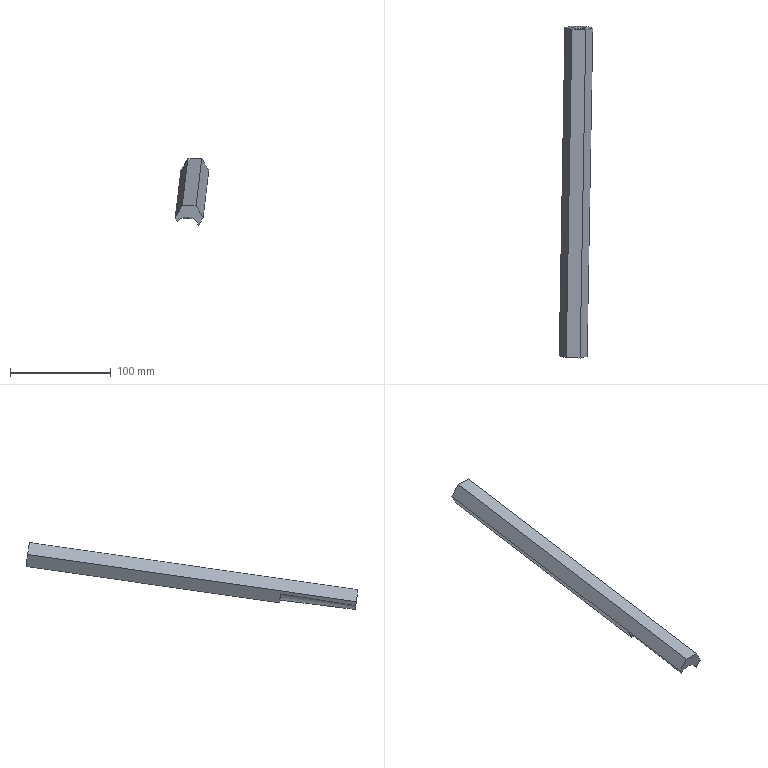Component | NX | HEX_STEEL | 1 solid | 12 faces | box 33.33 x 330.25 x 66.52 mm | volume 143704 mm3 | plane 9 | cylinder 2 | cone 1 | commonest cylinder face diameters 14 x1 25 x1
STEP:
#1=CARTESIAN_POINT('',(0.,0.,0.));
#2=DIRECTION('',(0.,0.,1.));
#3=DIRECTION('',(1.,0.,0.));
#4=AXIS2_PLACEMENT_3D('',#1,#2,#3);
#5=CARTESIAN_POINT('',(1340.241,698.717,571.115));
#6=VERTEX_POINT('',#5);
#7=CARTESIAN_POINT('',(1333.313,700.539,559.253));
#8=VERTEX_POINT('',#7);
#9=CARTESIAN_POINT('',(1340.241,698.717,571.115));
#10=DIRECTION('',(-0.4999,0.1315,-0.856));
#11=VECTOR('',#10,1.);
#12=LINE('',#9,#11);
#13=CARTESIAN_POINT('',(1345.864,1025.32,618.005));
#14=DIRECTION('',(-0.8659,-0.05645,0.497));
#15=DIRECTION('',(0.4978,0.,0.8673));
#16=AXIS2_PLACEMENT_3D('',#13,#14,#15);
#17=PLANE('',#16);
#18=CARTESIAN_POINT('',(-43.467,-327.125));
#19=DIRECTION('',(-0.9913,0.1317));
#20=VECTOR('',#19,1.);
#21=LINE('',#18,#20);
#22=(GEOMETRIC_REPRESENTATION_CONTEXT(2)PARAMETRIC_REPRESENTATION_CONTEXT()REPRESENTATION_CONTEXT('',''));
#23=DEFINITIONAL_REPRESENTATION('',(#21),#22);
#24=PCURVE('',#17,#23);
#25=CARTESIAN_POINT('',(13.556,791.589,83.34));
#26=DIRECTION('',(-0.01704,-0.9897,-0.1421));
#27=DIRECTION('',(0.,0.1421,-0.9899));
#28=AXIS2_PLACEMENT_3D('',#25,#26,#27);
#29=PLANE('',#28);
#30=CARTESIAN_POINT('',(-496.022,1326.877));
#31=DIRECTION('',(0.866,-0.5));
#32=VECTOR('',#31,1.);
#33=LINE('',#30,#32);
#34=(GEOMETRIC_REPRESENTATION_CONTEXT(2)PARAMETRIC_REPRESENTATION_CONTEXT()REPRESENTATION_CONTEXT('',''));
#35=DEFINITIONAL_REPRESENTATION('',(#33),#34);
#36=PCURVE('',#29,#35);
#37=SURFACE_CURVE('',#12,(#24,#36),.PCURVE_S1.);
#38=EDGE_CURVE('',#6,#8,#37,.T.);
#39=ORIENTED_EDGE('',*,*,#38,.F.);
#40=CARTESIAN_POINT('',(1345.864,1025.32,618.005));
#41=VERTEX_POINT('',#40);
#42=CARTESIAN_POINT('',(1345.864,1025.32,618.005));
#43=DIRECTION('',(-0.01704,-0.9897,-0.1421));
#44=VECTOR('',#43,1.);
#45=LINE('',#42,#44);
#46=CARTESIAN_POINT('',(0.,0.));
#47=DIRECTION('',(-0.1317,-0.9913));
#48=VECTOR('',#47,1.);
#49=LINE('',#46,#48);
#50=(GEOMETRIC_REPRESENTATION_CONTEXT(2)PARAMETRIC_REPRESENTATION_CONTEXT()REPRESENTATION_CONTEXT('',''));
#51=DEFINITIONAL_REPRESENTATION('',(#49),#50);
#52=PCURVE('',#17,#51);
#53=CARTESIAN_POINT('',(1359.718,1025.087,617.972));
#54=DIRECTION('',(0.,-0.1421,0.9899));
#55=DIRECTION('',(-0.,-0.9899,-0.1421));
#56=AXIS2_PLACEMENT_3D('',#53,#54,#55);
#57=PLANE('',#56);
#58=CARTESIAN_POINT('',(-0.2361,-13.854));
#59=DIRECTION('',(0.9999,-0.01704));
#60=VECTOR('',#59,1.);
#61=LINE('',#58,#60);
#62=(GEOMETRIC_REPRESENTATION_CONTEXT(2)PARAMETRIC_REPRESENTATION_CONTEXT()REPRESENTATION_CONTEXT('',''));
#63=DEFINITIONAL_REPRESENTATION('',(#61),#62);
#64=PCURVE('',#57,#63);
#65=SURFACE_CURVE('',#45,(#52,#64),.PCURVE_S1.);
#66=EDGE_CURVE('',#41,#6,#65,.T.);
#67=ORIENTED_EDGE('',*,*,#66,.F.);
#68=CARTESIAN_POINT('',(1338.937,1027.142,606.144));
#69=VERTEX_POINT('',#68);
#70=CARTESIAN_POINT('',(1345.864,1025.32,618.005));
#71=DIRECTION('',(-0.4999,0.1315,-0.856));
#72=VECTOR('',#71,1.);
#73=LINE('',#70,#72);
#74=CARTESIAN_POINT('',(0.,0.));
#75=DIRECTION('',(-0.9913,0.1317));
#76=VECTOR('',#75,1.);
#77=LINE('',#74,#76);
#78=(GEOMETRIC_REPRESENTATION_CONTEXT(2)PARAMETRIC_REPRESENTATION_CONTEXT()REPRESENTATION_CONTEXT('',''));
#79=DEFINITIONAL_REPRESENTATION('',(#77),#78);
#80=PCURVE('',#17,#79);
#81=CARTESIAN_POINT('',(19.179,1118.192,130.231));
#82=DIRECTION('',(-0.01704,-0.9897,-0.1421));
#83=DIRECTION('',(0.,0.1421,-0.9899));
#84=AXIS2_PLACEMENT_3D('',#81,#82,#83);
#85=PLANE('',#84);
#86=CARTESIAN_POINT('',(-496.022,1326.877));
#87=DIRECTION('',(0.866,-0.5));
#88=VECTOR('',#87,1.);
#89=LINE('',#86,#88);
#90=(GEOMETRIC_REPRESENTATION_CONTEXT(2)PARAMETRIC_REPRESENTATION_CONTEXT()REPRESENTATION_CONTEXT('',''));
#91=DEFINITIONAL_REPRESENTATION('',(#89),#90);
#92=PCURVE('',#85,#91);
#93=SURFACE_CURVE('',#73,(#80,#92),.PCURVE_S1.);
#94=EDGE_CURVE('',#41,#69,#93,.T.);
#95=ORIENTED_EDGE('',*,*,#94,.T.);
#96=CARTESIAN_POINT('',(1338.937,1027.142,606.144));
#97=DIRECTION('',(-0.01704,-0.9897,-0.1421));
#98=VECTOR('',#97,1.);
#99=LINE('',#96,#98);
#100=CARTESIAN_POINT('',(-13.736,1.825));
#101=DIRECTION('',(-0.1317,-0.9913));
#102=VECTOR('',#101,1.);
#103=LINE('',#100,#102);
#104=(GEOMETRIC_REPRESENTATION_CONTEXT(2)PARAMETRIC_REPRESENTATION_CONTEXT()REPRESENTATION_CONTEXT('',''));
#105=DEFINITIONAL_REPRESENTATION('',(#103),#104);
#106=PCURVE('',#17,#105);
#107=CARTESIAN_POINT('',(1338.937,1027.142,606.144));
#108=DIRECTION('',(-0.8659,0.08566,-0.4928));
#109=DIRECTION('',(-0.4946,0.,0.8691));
#110=AXIS2_PLACEMENT_3D('',#107,#108,#109);
#111=PLANE('',#110);
#112=CARTESIAN_POINT('',(0.,0.));
#113=DIRECTION('',(-0.1151,-0.9934));
#114=VECTOR('',#113,1.);
#115=LINE('',#112,#114);
#116=(GEOMETRIC_REPRESENTATION_CONTEXT(2)PARAMETRIC_REPRESENTATION_CONTEXT()REPRESENTATION_CONTEXT('',''));
#117=DEFINITIONAL_REPRESENTATION('',(#115),#116);
#118=PCURVE('',#111,#117);
#119=SURFACE_CURVE('',#99,(#106,#118),.PCURVE_S1.);
#120=EDGE_CURVE('',#69,#8,#119,.T.);
#121=ORIENTED_EDGE('',*,*,#120,.T.);
#122=EDGE_LOOP('',(#39,#67,#95,#121));
#123=FACE_BOUND('',#122,.T.);
#124=ADVANCED_FACE('',(#123),#17,.T.);
#125=CARTESIAN_POINT('',(1336.24,775.365,567.118));
#126=VERTEX_POINT('',#125);
#127=CARTESIAN_POINT('',(1341.524,776.666,558.06));
#128=VERTEX_POINT('',#127);
#129=CARTESIAN_POINT('',(1335.68,775.228,568.077));
#130=DIRECTION('',(0.5001,0.1231,-0.8572));
#131=VECTOR('',#130,1.);
#132=LINE('',#129,#131);
#133=CARTESIAN_POINT('',(-31.473,-252.844));
#134=DIRECTION('',(-0.9923,0.1235));
#135=VECTOR('',#134,1.);
#136=LINE('',#133,#135);
#137=(GEOMETRIC_REPRESENTATION_CONTEXT(2)PARAMETRIC_REPRESENTATION_CONTEXT()REPRESENTATION_CONTEXT('',''));
#138=DEFINITIONAL_REPRESENTATION('',(#136),#137);
#139=PCURVE('',#111,#138);
#140=CARTESIAN_POINT('',(1344.754,776.666,558.06));
#141=DIRECTION('',(0.,0.9899,0.1421));
#142=DIRECTION('',(0.,-0.1421,0.9899));
#143=AXIS2_PLACEMENT_3D('',#140,#141,#142);
#144=PLANE('',#143);
#145=CARTESIAN_POINT('',(10.12,-9.074));
#146=DIRECTION('',(-0.866,0.5001));
#147=VECTOR('',#146,1.);
#148=LINE('',#145,#147);
#149=(GEOMETRIC_REPRESENTATION_CONTEXT(2)PARAMETRIC_REPRESENTATION_CONTEXT()REPRESENTATION_CONTEXT('',''));
#150=DEFINITIONAL_REPRESENTATION('',(#148),#149);
#151=PCURVE('',#144,#150);
#152=SURFACE_CURVE('',#132,(#139,#151),.PCURVE_S1.);
#153=EDGE_CURVE('',#126,#128,#152,.T.);
#154=ORIENTED_EDGE('',*,*,#153,.F.);
#155=CARTESIAN_POINT('',(1335.433,701.025,555.614));
#156=VERTEX_POINT('',#155);
#157=CARTESIAN_POINT('',(1344.754,964.276,584.995));
#158=DIRECTION('',(-0.8659,0.08566,-0.4928));
#159=DIRECTION('',(0.01278,0.9887,0.1494));
#160=AXIS2_PLACEMENT_3D('',#157,#158,#159);
#161=ELLIPSE('',#160,847.024,12.5);
#162=CARTESIAN_POINT('',(-21.258,-63.098));
#163=DIRECTION('',(0.1235,0.9923));
#164=AXIS2_PLACEMENT_2D('',#162,#163);
#165=ELLIPSE('',#164,847.024,12.5);
#166=(GEOMETRIC_REPRESENTATION_CONTEXT(2)PARAMETRIC_REPRESENTATION_CONTEXT()REPRESENTATION_CONTEXT('',''));
#167=DEFINITIONAL_REPRESENTATION('',(#165),#166);
#168=PCURVE('',#111,#167);
#169=CARTESIAN_POINT('',(1344.754,657.884,541.006));
#170=DIRECTION('',(0.,0.9899,0.1421));
#171=DIRECTION('',(1.,0.,0.));
#172=AXIS2_PLACEMENT_3D('',#169,#170,#171);
#173=CYLINDRICAL_SURFACE('',#172,12.5);
#174=CARTESIAN_POINT('',(3.871,44.78));
#175=CARTESIAN_POINT('',(3.872,45.904));
#176=CARTESIAN_POINT('',(3.875,48.154));
#177=CARTESIAN_POINT('',(3.879,51.534));
#178=CARTESIAN_POINT('',(3.883,54.918));
#179=CARTESIAN_POINT('',(3.888,58.306));
#180=CARTESIAN_POINT('',(3.892,61.699));
#181=CARTESIAN_POINT('',(3.896,65.097));
#182=CARTESIAN_POINT('',(3.9,68.499));
#183=CARTESIAN_POINT('',(3.904,71.905));
#184=CARTESIAN_POINT('',(3.909,75.315));
#185=CARTESIAN_POINT('',(3.913,78.729));
#186=CARTESIAN_POINT('',(3.917,82.147));
#187=CARTESIAN_POINT('',(3.921,85.57));
#188=CARTESIAN_POINT('',(3.925,88.996));
#189=CARTESIAN_POINT('',(3.929,92.426));
#190=CARTESIAN_POINT('',(3.934,95.86));
#191=CARTESIAN_POINT('',(3.938,99.298));
#192=CARTESIAN_POINT('',(3.942,102.739));
#193=CARTESIAN_POINT('',(3.946,106.184));
#194=CARTESIAN_POINT('',(3.95,109.633));
#195=CARTESIAN_POINT('',(3.955,113.085));
#196=CARTESIAN_POINT('',(3.959,116.54));
#197=CARTESIAN_POINT('',(3.962,118.846));
#198=CARTESIAN_POINT('',(3.963,120.));
#199=B_SPLINE_CURVE_WITH_KNOTS('',3,(#174,#175,#176,#177,#178,#179,#180,#181,#182,#183,#184,#185,#186,#187,#188,#189,#190,#191,#192,#193,#194,#195,#196,#197,#198),.UNSPECIFIED.,.F.,.F.,(4,1,1,1,1,1,1,1,1,1,1,1,1,1,1,1,1,1,1,1,1,1,4),(4.394,4.399,4.403,4.407,4.411,4.415,4.42,4.424,4.428,4.432,4.436,4.441,4.445,4.449,4.453,4.457,4.462,4.466,4.47,4.474,4.478,4.482,4.487),.QUASI_UNIFORM_KNOTS.);
#200=(GEOMETRIC_REPRESENTATION_CONTEXT(2)PARAMETRIC_REPRESENTATION_CONTEXT()REPRESENTATION_CONTEXT('',''));
#201=DEFINITIONAL_REPRESENTATION('',(#199),#200);
#202=PCURVE('',#173,#201);
#203=SURFACE_CURVE('',#161,(#168,#202),.PCURVE_S1.);
#204=EDGE_CURVE('',#156,#126,#203,.T.);
#205=ORIENTED_EDGE('',*,*,#204,.F.);
#206=CARTESIAN_POINT('',(1333.313,700.539,559.253));
#207=DIRECTION('',(0.4999,0.1146,-0.8584));
#208=VECTOR('',#207,1.);
#209=LINE('',#206,#208);
#210=CARTESIAN_POINT('',(-37.97,-327.808));
#211=DIRECTION('',(-0.9934,0.1151));
#212=VECTOR('',#211,1.);
#213=LINE('',#210,#212);
#214=(GEOMETRIC_REPRESENTATION_CONTEXT(2)PARAMETRIC_REPRESENTATION_CONTEXT()REPRESENTATION_CONTEXT('',''));
#215=DEFINITIONAL_REPRESENTATION('',(#213),#214);
#216=PCURVE('',#111,#215);
#217=CARTESIAN_POINT('',(-484.022,1319.949));
#218=DIRECTION('',(0.866,0.5));
#219=VECTOR('',#218,1.);
#220=LINE('',#217,#219);
#221=(GEOMETRIC_REPRESENTATION_CONTEXT(2)PARAMETRIC_REPRESENTATION_CONTEXT()REPRESENTATION_CONTEXT('',''));
#222=DEFINITIONAL_REPRESENTATION('',(#220),#221);
#223=PCURVE('',#29,#222);
#224=SURFACE_CURVE('',#209,(#216,#223),.PCURVE_S1.);
#225=EDGE_CURVE('',#8,#156,#224,.T.);
#226=ORIENTED_EDGE('',*,*,#225,.F.);
#227=ORIENTED_EDGE('',*,*,#120,.F.);
#228=CARTESIAN_POINT('',(1345.864,1028.731,594.249));
#229=VERTEX_POINT('',#228);
#230=CARTESIAN_POINT('',(1338.937,1027.142,606.144));
#231=DIRECTION('',(0.4999,0.1146,-0.8584));
#232=VECTOR('',#231,1.);
#233=LINE('',#230,#232);
#234=CARTESIAN_POINT('',(0.,0.));
#235=DIRECTION('',(-0.9934,0.1151));
#236=VECTOR('',#235,1.);
#237=LINE('',#234,#236);
#238=(GEOMETRIC_REPRESENTATION_CONTEXT(2)PARAMETRIC_REPRESENTATION_CONTEXT()REPRESENTATION_CONTEXT('',''));
#239=DEFINITIONAL_REPRESENTATION('',(#237),#238);
#240=PCURVE('',#111,#239);
#241=CARTESIAN_POINT('',(-484.022,1319.949));
#242=DIRECTION('',(0.866,0.5));
#243=VECTOR('',#242,1.);
#244=LINE('',#241,#243);
#245=(GEOMETRIC_REPRESENTATION_CONTEXT(2)PARAMETRIC_REPRESENTATION_CONTEXT()REPRESENTATION_CONTEXT('',''));
#246=DEFINITIONAL_REPRESENTATION('',(#244),#245);
#247=PCURVE('',#85,#246);
#248=SURFACE_CURVE('',#233,(#240,#247),.PCURVE_S1.);
#249=EDGE_CURVE('',#69,#229,#248,.T.);
#250=ORIENTED_EDGE('',*,*,#249,.T.);
#251=CARTESIAN_POINT('',(1345.864,1028.731,594.249));
#252=DIRECTION('',(-0.01704,-0.9897,-0.1421));
#253=VECTOR('',#252,1.);
#254=LINE('',#251,#253);
#255=CARTESIAN_POINT('',(-13.764,1.594));
#256=DIRECTION('',(-0.1151,-0.9934));
#257=VECTOR('',#256,1.);
#258=LINE('',#255,#257);
#259=(GEOMETRIC_REPRESENTATION_CONTEXT(2)PARAMETRIC_REPRESENTATION_CONTEXT()REPRESENTATION_CONTEXT('',''));
#260=DEFINITIONAL_REPRESENTATION('',(#258),#259);
#261=PCURVE('',#111,#260);
#262=CARTESIAN_POINT('',(1345.864,1028.731,594.249));
#263=DIRECTION('',(-0.,0.1421,-0.9899));
#264=DIRECTION('',(0.,0.9899,0.1421));
#265=AXIS2_PLACEMENT_3D('',#262,#263,#264);
#266=PLANE('',#265);
#267=CARTESIAN_POINT('',(0.,0.));
#268=DIRECTION('',(-0.9999,-0.01704));
#269=VECTOR('',#268,1.);
#270=LINE('',#267,#269);
#271=(GEOMETRIC_REPRESENTATION_CONTEXT(2)PARAMETRIC_REPRESENTATION_CONTEXT()REPRESENTATION_CONTEXT('',''));
#272=DEFINITIONAL_REPRESENTATION('',(#270),#271);
#273=PCURVE('',#266,#272);
#274=SURFACE_CURVE('',#254,(#261,#273),.PCURVE_S1.);
#275=EDGE_CURVE('',#229,#128,#274,.T.);
#276=ORIENTED_EDGE('',*,*,#275,.T.);
#277=EDGE_LOOP('',(#154,#205,#226,#227,#250,#276));
#278=FACE_BOUND('',#277,.T.);
#279=ADVANCED_FACE('',(#278),#111,.T.);
#280=CARTESIAN_POINT('',(1355.382,776.666,558.06));
#281=VERTEX_POINT('',#280);
#282=CARTESIAN_POINT('',(1345.864,776.666,558.06));
#283=DIRECTION('',(1.,0.,-0.));
#284=VECTOR('',#283,1.);
#285=LINE('',#282,#284);
#286=CARTESIAN_POINT('',(-254.65,-0.));
#287=DIRECTION('',(-0.,1.));
#288=VECTOR('',#287,1.);
#289=LINE('',#286,#288);
#290=(GEOMETRIC_REPRESENTATION_CONTEXT(2)PARAMETRIC_REPRESENTATION_CONTEXT()REPRESENTATION_CONTEXT('',''));
#291=DEFINITIONAL_REPRESENTATION('',(#289),#290);
#292=PCURVE('',#266,#291);
#293=CARTESIAN_POINT('',(0.,1.11));
#294=DIRECTION('',(-0.,1.));
#295=VECTOR('',#294,1.);
#296=LINE('',#293,#295);
#297=(GEOMETRIC_REPRESENTATION_CONTEXT(2)PARAMETRIC_REPRESENTATION_CONTEXT()REPRESENTATION_CONTEXT('',''));
#298=DEFINITIONAL_REPRESENTATION('',(#296),#297);
#299=PCURVE('',#144,#298);
#300=SURFACE_CURVE('',#285,(#292,#299),.PCURVE_S1.);
#301=EDGE_CURVE('',#128,#281,#300,.T.);
#302=ORIENTED_EDGE('',*,*,#301,.F.);
#303=ORIENTED_EDGE('',*,*,#275,.F.);
#304=CARTESIAN_POINT('',(1359.718,1028.497,594.215));
#305=VERTEX_POINT('',#304);
#306=CARTESIAN_POINT('',(1345.864,1028.731,594.249));
#307=DIRECTION('',(0.9999,-0.01687,-0.002422));
#308=VECTOR('',#307,1.);
#309=LINE('',#306,#308);
#310=CARTESIAN_POINT('',(0.,0.));
#311=DIRECTION('',(-0.01704,0.9999));
#312=VECTOR('',#311,1.);
#313=LINE('',#310,#312);
#314=(GEOMETRIC_REPRESENTATION_CONTEXT(2)PARAMETRIC_REPRESENTATION_CONTEXT()REPRESENTATION_CONTEXT('',''));
#315=DEFINITIONAL_REPRESENTATION('',(#313),#314);
#316=PCURVE('',#266,#315);
#317=CARTESIAN_POINT('',(-472.022,1326.877));
#318=DIRECTION('',(0.,1.));
#319=VECTOR('',#318,1.);
#320=LINE('',#317,#319);
#321=(GEOMETRIC_REPRESENTATION_CONTEXT(2)PARAMETRIC_REPRESENTATION_CONTEXT()REPRESENTATION_CONTEXT('',''));
#322=DEFINITIONAL_REPRESENTATION('',(#320),#321);
#323=PCURVE('',#85,#322);
#324=SURFACE_CURVE('',#309,(#316,#323),.PCURVE_S1.);
#325=EDGE_CURVE('',#229,#305,#324,.T.);
#326=ORIENTED_EDGE('',*,*,#325,.T.);
#327=CARTESIAN_POINT('',(1359.718,1028.497,594.215));
#328=DIRECTION('',(-0.01704,-0.9897,-0.1421));
#329=VECTOR('',#328,1.);
#330=LINE('',#327,#329);
#331=CARTESIAN_POINT('',(-0.2361,13.854));
#332=DIRECTION('',(-0.9999,-0.01704));
#333=VECTOR('',#332,1.);
#334=LINE('',#331,#333);
#335=(GEOMETRIC_REPRESENTATION_CONTEXT(2)PARAMETRIC_REPRESENTATION_CONTEXT()REPRESENTATION_CONTEXT('',''));
#336=DEFINITIONAL_REPRESENTATION('',(#334),#335);
#337=PCURVE('',#266,#336);
#338=CARTESIAN_POINT('',(1359.718,1028.497,594.215));
#339=DIRECTION('',(0.8659,0.05645,-0.497));
#340=DIRECTION('',(-0.4978,0.,-0.8673));
#341=AXIS2_PLACEMENT_3D('',#338,#339,#340);
#342=PLANE('',#341);
#343=CARTESIAN_POINT('',(0.,0.));
#344=DIRECTION('',(0.1317,-0.9913));
#345=VECTOR('',#344,1.);
#346=LINE('',#343,#345);
#347=(GEOMETRIC_REPRESENTATION_CONTEXT(2)PARAMETRIC_REPRESENTATION_CONTEXT()REPRESENTATION_CONTEXT('',''));
#348=DEFINITIONAL_REPRESENTATION('',(#346),#347);
#349=PCURVE('',#342,#348);
#350=SURFACE_CURVE('',#330,(#337,#349),.PCURVE_S1.);
#351=EDGE_CURVE('',#305,#281,#350,.T.);
#352=ORIENTED_EDGE('',*,*,#351,.T.);
#353=EDGE_LOOP('',(#302,#303,#326,#352));
#354=FACE_BOUND('',#353,.T.);
#355=ADVANCED_FACE('',(#354),#266,.T.);
#356=CARTESIAN_POINT('',(1356.954,776.279,560.754));
#357=VERTEX_POINT('',#356);
#358=CARTESIAN_POINT('',(1356.467,776.399,559.918));
#359=DIRECTION('',(0.5001,-0.1231,0.8572));
#360=VECTOR('',#359,1.);
#361=LINE('',#358,#360);
#362=CARTESIAN_POINT('',(31.364,-252.501));
#363=DIRECTION('',(-0.9924,-0.1233));
#364=VECTOR('',#363,1.);
#365=LINE('',#362,#364);
#366=(GEOMETRIC_REPRESENTATION_CONTEXT(2)PARAMETRIC_REPRESENTATION_CONTEXT()REPRESENTATION_CONTEXT('',''));
#367=DEFINITIONAL_REPRESENTATION('',(#365),#366);
#368=PCURVE('',#342,#367);
#369=CARTESIAN_POINT('',(1.878,11.712));
#370=DIRECTION('',(0.866,0.5001));
#371=VECTOR('',#370,1.);
#372=LINE('',#369,#371);
#373=(GEOMETRIC_REPRESENTATION_CONTEXT(2)PARAMETRIC_REPRESENTATION_CONTEXT()REPRESENTATION_CONTEXT('',''));
#374=DEFINITIONAL_REPRESENTATION('',(#372),#373);
#375=PCURVE('',#144,#374);
#376=SURFACE_CURVE('',#361,(#368,#375),.PCURVE_S1.);
#377=EDGE_CURVE('',#281,#357,#376,.T.);
#378=ORIENTED_EDGE('',*,*,#377,.F.);
#379=ORIENTED_EDGE('',*,*,#351,.F.);
#380=CARTESIAN_POINT('',(1366.646,1026.675,606.077));
#381=VERTEX_POINT('',#380);
#382=CARTESIAN_POINT('',(1359.718,1028.497,594.215));
#383=DIRECTION('',(0.4999,-0.1315,0.856));
#384=VECTOR('',#383,1.);
#385=LINE('',#382,#384);
#386=CARTESIAN_POINT('',(0.,0.));
#387=DIRECTION('',(-0.9913,-0.1317));
#388=VECTOR('',#387,1.);
#389=LINE('',#386,#388);
#390=(GEOMETRIC_REPRESENTATION_CONTEXT(2)PARAMETRIC_REPRESENTATION_CONTEXT()REPRESENTATION_CONTEXT('',''));
#391=DEFINITIONAL_REPRESENTATION('',(#389),#390);
#392=PCURVE('',#342,#391);
#393=CARTESIAN_POINT('',(-472.022,1340.734));
#394=DIRECTION('',(-0.866,0.5));
#395=VECTOR('',#394,1.);
#396=LINE('',#393,#395);
#397=(GEOMETRIC_REPRESENTATION_CONTEXT(2)PARAMETRIC_REPRESENTATION_CONTEXT()REPRESENTATION_CONTEXT('',''));
#398=DEFINITIONAL_REPRESENTATION('',(#396),#397);
#399=PCURVE('',#85,#398);
#400=SURFACE_CURVE('',#385,(#392,#399),.PCURVE_S1.);
#401=EDGE_CURVE('',#305,#381,#400,.T.);
#402=ORIENTED_EDGE('',*,*,#401,.T.);
#403=CARTESIAN_POINT('',(1361.022,700.072,559.186));
#404=VERTEX_POINT('',#403);
#405=CARTESIAN_POINT('',(1366.646,1026.675,606.077));
#406=DIRECTION('',(-0.01704,-0.9897,-0.1421));
#407=VECTOR('',#406,1.);
#408=LINE('',#405,#407);
#409=CARTESIAN_POINT('',(-13.736,-1.825));
#410=DIRECTION('',(0.1317,-0.9913));
#411=VECTOR('',#410,1.);
#412=LINE('',#409,#411);
#413=(GEOMETRIC_REPRESENTATION_CONTEXT(2)PARAMETRIC_REPRESENTATION_CONTEXT()REPRESENTATION_CONTEXT('',''));
#414=DEFINITIONAL_REPRESENTATION('',(#412),#413);
#415=PCURVE('',#342,#414);
#416=CARTESIAN_POINT('',(1366.646,1026.675,606.077));
#417=DIRECTION('',(0.8659,-0.08566,0.4928));
#418=DIRECTION('',(0.4946,0.,-0.8691));
#419=AXIS2_PLACEMENT_3D('',#416,#417,#418);
#420=PLANE('',#419);
#421=CARTESIAN_POINT('',(0.,0.));
#422=DIRECTION('',(0.1151,-0.9934));
#423=VECTOR('',#422,1.);
#424=LINE('',#421,#423);
#425=(GEOMETRIC_REPRESENTATION_CONTEXT(2)PARAMETRIC_REPRESENTATION_CONTEXT()REPRESENTATION_CONTEXT('',''));
#426=DEFINITIONAL_REPRESENTATION('',(#424),#425);
#427=PCURVE('',#420,#426);
#428=SURFACE_CURVE('',#408,(#415,#427),.PCURVE_S1.);
#429=EDGE_CURVE('',#381,#404,#428,.T.);
#430=ORIENTED_EDGE('',*,*,#429,.T.);
#431=CARTESIAN_POINT('',(1356.524,701.255,551.485));
#432=VERTEX_POINT('',#431);
#433=CARTESIAN_POINT('',(1354.095,701.894,547.325));
#434=DIRECTION('',(0.4999,-0.1315,0.856));
#435=VECTOR('',#434,1.);
#436=LINE('',#433,#435);
#437=CARTESIAN_POINT('',(43.467,-327.125));
#438=DIRECTION('',(-0.9913,-0.1317));
#439=VECTOR('',#438,1.);
#440=LINE('',#437,#439);
#441=(GEOMETRIC_REPRESENTATION_CONTEXT(2)PARAMETRIC_REPRESENTATION_CONTEXT()REPRESENTATION_CONTEXT('',''));
#442=DEFINITIONAL_REPRESENTATION('',(#440),#441);
#443=PCURVE('',#342,#442);
#444=CARTESIAN_POINT('',(-472.022,1340.734));
#445=DIRECTION('',(-0.866,0.5));
#446=VECTOR('',#445,1.);
#447=LINE('',#444,#446);
#448=(GEOMETRIC_REPRESENTATION_CONTEXT(2)PARAMETRIC_REPRESENTATION_CONTEXT()REPRESENTATION_CONTEXT('',''));
#449=DEFINITIONAL_REPRESENTATION('',(#447),#448);
#450=PCURVE('',#29,#449);
#451=SURFACE_CURVE('',#436,(#443,#450),.PCURVE_S1.);
#452=EDGE_CURVE('',#432,#404,#451,.T.);
#453=ORIENTED_EDGE('',*,*,#452,.F.);
#454=CARTESIAN_POINT('',(1344.754,159.386,469.437));
#455=DIRECTION('',(0.8659,0.05645,-0.497));
#456=DIRECTION('',(0.01278,0.9908,0.1348));
#457=AXIS2_PLACEMENT_3D('',#454,#455,#456);
#458=ELLIPSE('',#457,847.024,12.5);
#459=CARTESIAN_POINT('',(115.667,-870.499));
#460=DIRECTION('',(-0.1233,0.9924));
#461=AXIS2_PLACEMENT_2D('',#459,#460);
#462=ELLIPSE('',#461,847.024,12.5);
#463=(GEOMETRIC_REPRESENTATION_CONTEXT(2)PARAMETRIC_REPRESENTATION_CONTEXT()REPRESENTATION_CONTEXT('',''));
#464=DEFINITIONAL_REPRESENTATION('',(#462),#463);
#465=PCURVE('',#342,#464);
#466=CARTESIAN_POINT('',(6.064,120.));
#467=CARTESIAN_POINT('',(6.062,118.924));
#468=CARTESIAN_POINT('',(6.058,116.767));
#469=CARTESIAN_POINT('',(6.052,113.511));
#470=CARTESIAN_POINT('',(6.047,110.235));
#471=CARTESIAN_POINT('',(6.041,106.94));
#472=CARTESIAN_POINT('',(6.036,103.626));
#473=CARTESIAN_POINT('',(6.03,100.292));
#474=CARTESIAN_POINT('',(6.024,96.939));
#475=CARTESIAN_POINT('',(6.019,93.567));
#476=CARTESIAN_POINT('',(6.013,90.176));
#477=CARTESIAN_POINT('',(6.007,86.767));
#478=CARTESIAN_POINT('',(6.002,83.338));
#479=CARTESIAN_POINT('',(5.996,79.892));
#480=CARTESIAN_POINT('',(5.99,76.426));
#481=CARTESIAN_POINT('',(5.985,72.942));
#482=CARTESIAN_POINT('',(5.979,69.44));
#483=CARTESIAN_POINT('',(5.974,65.92));
#484=CARTESIAN_POINT('',(5.968,62.382));
#485=CARTESIAN_POINT('',(5.962,58.825));
#486=CARTESIAN_POINT('',(5.957,55.251));
#487=CARTESIAN_POINT('',(5.951,51.659));
#488=CARTESIAN_POINT('',(5.945,48.05));
#489=CARTESIAN_POINT('',(5.942,45.632));
#490=CARTESIAN_POINT('',(5.94,44.42));
#491=B_SPLINE_CURVE_WITH_KNOTS('',3,(#466,#467,#468,#469,#470,#471,#472,#473,#474,#475,#476,#477,#478,#479,#480,#481,#482,#483,#484,#485,#486,#487,#488,#489,#490),.UNSPECIFIED.,.F.,.F.,(4,1,1,1,1,1,1,1,1,1,1,1,1,1,1,1,1,1,1,1,1,1,4),(0.7432,0.7488,0.7544,0.7601,0.7657,0.7713,0.777,0.7826,0.7882,0.7939,0.7995,0.8051,0.8108,0.8164,0.822,0.8276,0.8333,0.8389,0.8445,0.8502,0.8558,0.8614,0.8671),.QUASI_UNIFORM_KNOTS.);
#492=(GEOMETRIC_REPRESENTATION_CONTEXT(2)PARAMETRIC_REPRESENTATION_CONTEXT()REPRESENTATION_CONTEXT('',''));
#493=DEFINITIONAL_REPRESENTATION('',(#491),#492);
#494=PCURVE('',#173,#493);
#495=SURFACE_CURVE('',#458,(#465,#494),.PCURVE_S1.);
#496=EDGE_CURVE('',#357,#432,#495,.T.);
#497=ORIENTED_EDGE('',*,*,#496,.F.);
#498=EDGE_LOOP('',(#378,#379,#402,#430,#453,#497));
#499=FACE_BOUND('',#498,.T.);
#500=ADVANCED_FACE('',(#499),#342,.T.);
#501=CARTESIAN_POINT('',(1354.095,698.483,571.081));
#502=VERTEX_POINT('',#501);
#503=CARTESIAN_POINT('',(1361.022,700.072,559.186));
#504=DIRECTION('',(-0.4999,-0.1146,0.8584));
#505=VECTOR('',#504,1.);
#506=LINE('',#503,#505);
#507=CARTESIAN_POINT('',(37.97,-327.808));
#508=DIRECTION('',(-0.9934,-0.1151));
#509=VECTOR('',#508,1.);
#510=LINE('',#507,#509);
#511=(GEOMETRIC_REPRESENTATION_CONTEXT(2)PARAMETRIC_REPRESENTATION_CONTEXT()REPRESENTATION_CONTEXT('',''));
#512=DEFINITIONAL_REPRESENTATION('',(#510),#511);
#513=PCURVE('',#420,#512);
#514=CARTESIAN_POINT('',(-484.022,1347.662));
#515=DIRECTION('',(-0.866,-0.5));
#516=VECTOR('',#515,1.);
#517=LINE('',#514,#516);
#518=(GEOMETRIC_REPRESENTATION_CONTEXT(2)PARAMETRIC_REPRESENTATION_CONTEXT()REPRESENTATION_CONTEXT('',''));
#519=DEFINITIONAL_REPRESENTATION('',(#517),#518);
#520=PCURVE('',#29,#519);
#521=SURFACE_CURVE('',#506,(#513,#520),.PCURVE_S1.);
#522=EDGE_CURVE('',#404,#502,#521,.T.);
#523=ORIENTED_EDGE('',*,*,#522,.F.);
#524=ORIENTED_EDGE('',*,*,#429,.F.);
#525=CARTESIAN_POINT('',(1359.718,1025.087,617.972));
#526=VERTEX_POINT('',#525);
#527=CARTESIAN_POINT('',(1366.646,1026.675,606.077));
#528=DIRECTION('',(-0.4999,-0.1146,0.8584));
#529=VECTOR('',#528,1.);
#530=LINE('',#527,#529);
#531=CARTESIAN_POINT('',(0.,0.));
#532=DIRECTION('',(-0.9934,-0.1151));
#533=VECTOR('',#532,1.);
#534=LINE('',#531,#533);
#535=(GEOMETRIC_REPRESENTATION_CONTEXT(2)PARAMETRIC_REPRESENTATION_CONTEXT()REPRESENTATION_CONTEXT('',''));
#536=DEFINITIONAL_REPRESENTATION('',(#534),#535);
#537=PCURVE('',#420,#536);
#538=CARTESIAN_POINT('',(-484.022,1347.662));
#539=DIRECTION('',(-0.866,-0.5));
#540=VECTOR('',#539,1.);
#541=LINE('',#538,#540);
#542=(GEOMETRIC_REPRESENTATION_CONTEXT(2)PARAMETRIC_REPRESENTATION_CONTEXT()REPRESENTATION_CONTEXT('',''));
#543=DEFINITIONAL_REPRESENTATION('',(#541),#542);
#544=PCURVE('',#85,#543);
#545=SURFACE_CURVE('',#530,(#537,#544),.PCURVE_S1.);
#546=EDGE_CURVE('',#381,#526,#545,.T.);
#547=ORIENTED_EDGE('',*,*,#546,.T.);
#548=CARTESIAN_POINT('',(1359.718,1025.087,617.972));
#549=DIRECTION('',(-0.01704,-0.9897,-0.1421));
#550=VECTOR('',#549,1.);
#551=LINE('',#548,#550);
#552=CARTESIAN_POINT('',(-13.764,-1.594));
#553=DIRECTION('',(0.1151,-0.9934));
#554=VECTOR('',#553,1.);
#555=LINE('',#552,#554);
#556=(GEOMETRIC_REPRESENTATION_CONTEXT(2)PARAMETRIC_REPRESENTATION_CONTEXT()REPRESENTATION_CONTEXT('',''));
#557=DEFINITIONAL_REPRESENTATION('',(#555),#556);
#558=PCURVE('',#420,#557);
#559=CARTESIAN_POINT('',(0.,0.));
#560=DIRECTION('',(0.9999,-0.01704));
#561=VECTOR('',#560,1.);
#562=LINE('',#559,#561);
#563=(GEOMETRIC_REPRESENTATION_CONTEXT(2)PARAMETRIC_REPRESENTATION_CONTEXT()REPRESENTATION_CONTEXT('',''));
#564=DEFINITIONAL_REPRESENTATION('',(#562),#563);
#565=PCURVE('',#57,#564);
#566=SURFACE_CURVE('',#551,(#558,#565),.PCURVE_S1.);
#567=EDGE_CURVE('',#526,#502,#566,.T.);
#568=ORIENTED_EDGE('',*,*,#567,.T.);
#569=EDGE_LOOP('',(#523,#524,#547,#568));
#570=FACE_BOUND('',#569,.T.);
#571=ADVANCED_FACE('',(#570),#420,.T.);
#572=CARTESIAN_POINT('',(1354.095,698.483,571.081));
#573=DIRECTION('',(-0.9999,0.01687,0.002422));
#574=VECTOR('',#573,1.);
#575=LINE('',#572,#574);
#576=CARTESIAN_POINT('',(329.952,-5.623));
#577=DIRECTION('',(-0.01704,-0.9999));
#578=VECTOR('',#577,1.);
#579=LINE('',#576,#578);
#580=(GEOMETRIC_REPRESENTATION_CONTEXT(2)PARAMETRIC_REPRESENTATION_CONTEXT()REPRESENTATION_CONTEXT('',''));
#581=DEFINITIONAL_REPRESENTATION('',(#579),#580);
#582=PCURVE('',#57,#581);
#583=CARTESIAN_POINT('',(-496.022,1340.734));
#584=DIRECTION('',(-0.,-1.));
#585=VECTOR('',#584,1.);
#586=LINE('',#583,#585);
#587=(GEOMETRIC_REPRESENTATION_CONTEXT(2)PARAMETRIC_REPRESENTATION_CONTEXT()REPRESENTATION_CONTEXT('',''));
#588=DEFINITIONAL_REPRESENTATION('',(#586),#587);
#589=PCURVE('',#29,#588);
#590=SURFACE_CURVE('',#575,(#582,#589),.PCURVE_S1.);
#591=EDGE_CURVE('',#502,#6,#590,.T.);
#592=ORIENTED_EDGE('',*,*,#591,.F.);
#593=ORIENTED_EDGE('',*,*,#567,.F.);
#594=CARTESIAN_POINT('',(1359.718,1025.087,617.972));
#595=DIRECTION('',(-0.9999,0.01687,0.002422));
#596=VECTOR('',#595,1.);
#597=LINE('',#594,#596);
#598=CARTESIAN_POINT('',(0.,0.));
#599=DIRECTION('',(-0.01704,-0.9999));
#600=VECTOR('',#599,1.);
#601=LINE('',#598,#600);
#602=(GEOMETRIC_REPRESENTATION_CONTEXT(2)PARAMETRIC_REPRESENTATION_CONTEXT()REPRESENTATION_CONTEXT('',''));
#603=DEFINITIONAL_REPRESENTATION('',(#601),#602);
#604=PCURVE('',#57,#603);
#605=CARTESIAN_POINT('',(-496.022,1340.734));
#606=DIRECTION('',(-0.,-1.));
#607=VECTOR('',#606,1.);
#608=LINE('',#605,#607);
#609=(GEOMETRIC_REPRESENTATION_CONTEXT(2)PARAMETRIC_REPRESENTATION_CONTEXT()REPRESENTATION_CONTEXT('',''));
#610=DEFINITIONAL_REPRESENTATION('',(#608),#609);
#611=PCURVE('',#85,#610);
#612=SURFACE_CURVE('',#597,(#604,#611),.PCURVE_S1.);
#613=EDGE_CURVE('',#526,#41,#612,.T.);
#614=ORIENTED_EDGE('',*,*,#613,.T.);
#615=ORIENTED_EDGE('',*,*,#66,.T.);
#616=EDGE_LOOP('',(#592,#593,#614,#615));
#617=FACE_BOUND('',#616,.T.);
#618=ADVANCED_FACE('',(#617),#57,.T.);
#619=CARTESIAN_POINT('',(1352.791,1027.904,599.181));
#620=VERTEX_POINT('',#619);
#621=CARTESIAN_POINT('',(1352.791,1026.909,606.11));
#622=DIRECTION('',(-0.01704,-0.9897,-0.1421));
#623=DIRECTION('',(-0.,0.1421,-0.9899));
#624=AXIS2_PLACEMENT_3D('',#621,#622,#623);
#625=CIRCLE('',#624,7.);
#626=CARTESIAN_POINT('',(-484.022,1333.805));
#627=DIRECTION('',(1.,-0.));
#628=AXIS2_PLACEMENT_2D('',#626,#627);
#629=CIRCLE('',#628,7.);
#630=(GEOMETRIC_REPRESENTATION_CONTEXT(2)PARAMETRIC_REPRESENTATION_CONTEXT()REPRESENTATION_CONTEXT('',''));
#631=DEFINITIONAL_REPRESENTATION('',(#629),#630);
#632=PCURVE('',#85,#631);
#633=CARTESIAN_POINT('',(1352.791,1026.909,606.11));
#634=DIRECTION('',(-0.01704,-0.9897,-0.1421));
#635=DIRECTION('',(-0.,0.1421,-0.9899));
#636=AXIS2_PLACEMENT_3D('',#633,#634,#635);
#637=CYLINDRICAL_SURFACE('',#636,7.);
#638=CARTESIAN_POINT('',(0.,0.));
#639=DIRECTION('',(1.,0.));
#640=VECTOR('',#639,1.);
#641=LINE('',#638,#640);
#642=(GEOMETRIC_REPRESENTATION_CONTEXT(2)PARAMETRIC_REPRESENTATION_CONTEXT()REPRESENTATION_CONTEXT('',''));
#643=DEFINITIONAL_REPRESENTATION('',(#641),#642);
#644=PCURVE('',#637,#643);
#645=SURFACE_CURVE('',#625,(#632,#644),.PCURVE_S1.);
#646=EDGE_CURVE('',#620,#620,#645,.T.);
#647=ORIENTED_EDGE('',*,*,#646,.T.);
#648=EDGE_LOOP('',(#647));
#649=FACE_BOUND('',#648,.T.);
#650=ORIENTED_EDGE('',*,*,#94,.F.);
#651=ORIENTED_EDGE('',*,*,#613,.F.);
#652=ORIENTED_EDGE('',*,*,#546,.F.);
#653=ORIENTED_EDGE('',*,*,#401,.F.);
#654=ORIENTED_EDGE('',*,*,#325,.F.);
#655=ORIENTED_EDGE('',*,*,#249,.F.);
#656=EDGE_LOOP('',(#650,#651,#652,#653,#654,#655));
#657=FACE_BOUND('',#656,.T.);
#658=ADVANCED_FACE('',(#649,#657),#85,.F.);
#659=CARTESIAN_POINT('',(1344.754,702.052,547.347));
#660=DIRECTION('',(-0.01704,-0.9897,-0.1421));
#661=DIRECTION('',(-0.9999,0.01687,0.002422));
#662=AXIS2_PLACEMENT_3D('',#659,#660,#661);
#663=ELLIPSE('',#662,12.502,12.5);
#664=CARTESIAN_POINT('',(-472.022,1331.391));
#665=DIRECTION('',(0.,-1.));
#666=AXIS2_PLACEMENT_2D('',#664,#665);
#667=ELLIPSE('',#666,12.502,12.5);
#668=(GEOMETRIC_REPRESENTATION_CONTEXT(2)PARAMETRIC_REPRESENTATION_CONTEXT()REPRESENTATION_CONTEXT('',''));
#669=DEFINITIONAL_REPRESENTATION('',(#667),#668);
#670=PCURVE('',#29,#669);
#671=CARTESIAN_POINT('',(5.94,44.42));
#672=CARTESIAN_POINT('',(3.871,44.78));
#673=B_SPLINE_CURVE_WITH_KNOTS('',1,(#671,#672),.UNSPECIFIED.,.F.,.F.,(2,2),(3.485,5.554),.PIECEWISE_BEZIER_KNOTS.);
#674=(GEOMETRIC_REPRESENTATION_CONTEXT(2)PARAMETRIC_REPRESENTATION_CONTEXT()REPRESENTATION_CONTEXT('',''));
#675=DEFINITIONAL_REPRESENTATION('',(#673),#674);
#676=PCURVE('',#173,#675);
#677=SURFACE_CURVE('',#663,(#670,#676),.PCURVE_S1.);
#678=EDGE_CURVE('',#432,#156,#677,.T.);
#679=ORIENTED_EDGE('',*,*,#678,.F.);
#680=ORIENTED_EDGE('',*,*,#452,.T.);
#681=ORIENTED_EDGE('',*,*,#522,.T.);
#682=ORIENTED_EDGE('',*,*,#591,.T.);
#683=ORIENTED_EDGE('',*,*,#38,.T.);
#684=ORIENTED_EDGE('',*,*,#225,.T.);
#685=EDGE_LOOP('',(#679,#680,#681,#682,#683,#684));
#686=FACE_BOUND('',#685,.T.);
#687=ADVANCED_FACE('',(#686),#29,.T.);
#688=CARTESIAN_POINT('',(1352.144,988.305,607.64));
#689=VERTEX_POINT('',#688);
#690=CARTESIAN_POINT('',(1352.144,990.295,593.782));
#691=VERTEX_POINT('',#690);
#692=CARTESIAN_POINT('',(1352.144,989.3,600.711));
#693=DIRECTION('',(0.01704,0.9897,0.1421));
#694=DIRECTION('',(-0.,0.1421,-0.9899));
#695=AXIS2_PLACEMENT_3D('',#692,#693,#694);
#696=CIRCLE('',#695,7.);
#697=CARTESIAN_POINT('',(1352.144,989.3,600.711));
#698=DIRECTION('',(0.01704,0.9897,0.1421));
#699=DIRECTION('',(-0.,-0.1421,0.9899));
#700=AXIS2_PLACEMENT_3D('',#697,#698,#699);
#701=CONICAL_SURFACE('',#700,7.,1.047);
#702=CARTESIAN_POINT('',(-3.142,0.));
#703=DIRECTION('',(1.,0.));
#704=VECTOR('',#703,1.);
#705=LINE('',#702,#704);
#706=(GEOMETRIC_REPRESENTATION_CONTEXT(2)PARAMETRIC_REPRESENTATION_CONTEXT()REPRESENTATION_CONTEXT('',''));
#707=DEFINITIONAL_REPRESENTATION('',(#705),#706);
#708=PCURVE('',#701,#707);
#709=CARTESIAN_POINT('',(6.283,38.));
#710=DIRECTION('',(-1.,0.));
#711=VECTOR('',#710,1.);
#712=LINE('',#709,#711);
#713=(GEOMETRIC_REPRESENTATION_CONTEXT(2)PARAMETRIC_REPRESENTATION_CONTEXT()REPRESENTATION_CONTEXT('',''));
#714=DEFINITIONAL_REPRESENTATION('',(#712),#713);
#715=PCURVE('',#637,#714);
#716=SURFACE_CURVE('',#696,(#708,#715),.PCURVE_S1.);
#717=EDGE_CURVE('',#689,#691,#716,.T.);
#718=ORIENTED_EDGE('',*,*,#717,.F.);
#719=CARTESIAN_POINT('',(1352.075,985.3,600.136));
#720=VERTEX_POINT('',#719);
#721=CARTESIAN_POINT('',(1352.075,985.3,600.136));
#722=CARTESIAN_POINT('',(1352.144,988.305,607.64));
#723=B_SPLINE_CURVE_WITH_KNOTS('',1,(#721,#722),.UNSPECIFIED.,.F.,.F.,(2,2),(-8.083,0.),.PIECEWISE_BEZIER_KNOTS.);
#724=CARTESIAN_POINT('',(0.,0.));
#725=DIRECTION('',(0.,1.));
#726=VECTOR('',#725,1.);
#727=LINE('',#724,#726);
#728=(GEOMETRIC_REPRESENTATION_CONTEXT(2)PARAMETRIC_REPRESENTATION_CONTEXT()REPRESENTATION_CONTEXT('',''));
#729=DEFINITIONAL_REPRESENTATION('',(#727),#728);
#730=PCURVE('',#701,#729);
#731=CARTESIAN_POINT('',(6.283,0.));
#732=DIRECTION('',(0.,1.));
#733=VECTOR('',#732,1.);
#734=LINE('',#731,#733);
#735=(GEOMETRIC_REPRESENTATION_CONTEXT(2)PARAMETRIC_REPRESENTATION_CONTEXT()REPRESENTATION_CONTEXT('',''));
#736=DEFINITIONAL_REPRESENTATION('',(#734),#735);
#737=PCURVE('',#701,#736);
#738=SEAM_CURVE('',#723,(#730,#737),.PCURVE_S1.);
#739=EDGE_CURVE('',#720,#689,#738,.T.);
#740=ORIENTED_EDGE('',*,*,#739,.F.);
#741=ORIENTED_EDGE('',*,*,#739,.T.);
#742=CARTESIAN_POINT('',(1352.144,989.3,600.711));
#743=DIRECTION('',(0.01704,0.9897,0.1421));
#744=DIRECTION('',(-0.,0.1421,-0.9899));
#745=AXIS2_PLACEMENT_3D('',#742,#743,#744);
#746=CIRCLE('',#745,7.);
#747=CARTESIAN_POINT('',(3.142,0.));
#748=DIRECTION('',(1.,0.));
#749=VECTOR('',#748,1.);
#750=LINE('',#747,#749);
#751=(GEOMETRIC_REPRESENTATION_CONTEXT(2)PARAMETRIC_REPRESENTATION_CONTEXT()REPRESENTATION_CONTEXT('',''));
#752=DEFINITIONAL_REPRESENTATION('',(#750),#751);
#753=PCURVE('',#701,#752);
#754=CARTESIAN_POINT('',(6.283,38.));
#755=DIRECTION('',(-1.,0.));
#756=VECTOR('',#755,1.);
#757=LINE('',#754,#756);
#758=(GEOMETRIC_REPRESENTATION_CONTEXT(2)PARAMETRIC_REPRESENTATION_CONTEXT()REPRESENTATION_CONTEXT('',''));
#759=DEFINITIONAL_REPRESENTATION('',(#757),#758);
#760=PCURVE('',#637,#759);
#761=SURFACE_CURVE('',#746,(#753,#760),.PCURVE_S1.);
#762=EDGE_CURVE('',#691,#689,#761,.T.);
#763=ORIENTED_EDGE('',*,*,#762,.F.);
#764=EDGE_LOOP('',(#718,#740,#741,#763));
#765=FACE_BOUND('',#764,.F.);
#766=ADVANCED_FACE('',(#765),#701,.F.);
#767=ORIENTED_EDGE('',*,*,#717,.T.);
#768=CARTESIAN_POINT('',(1352.791,1027.904,599.181));
#769=CARTESIAN_POINT('',(1352.144,990.295,593.782));
#770=B_SPLINE_CURVE_WITH_KNOTS('',1,(#768,#769),.UNSPECIFIED.,.F.,.F.,(2,2),(0.,38.),.PIECEWISE_BEZIER_KNOTS.);
#771=CARTESIAN_POINT('',(0.,0.));
#772=DIRECTION('',(0.,1.));
#773=VECTOR('',#772,1.);
#774=LINE('',#771,#773);
#775=(GEOMETRIC_REPRESENTATION_CONTEXT(2)PARAMETRIC_REPRESENTATION_CONTEXT()REPRESENTATION_CONTEXT('',''));
#776=DEFINITIONAL_REPRESENTATION('',(#774),#775);
#777=PCURVE('',#637,#776);
#778=CARTESIAN_POINT('',(6.283,0.));
#779=DIRECTION('',(0.,1.));
#780=VECTOR('',#779,1.);
#781=LINE('',#778,#780);
#782=(GEOMETRIC_REPRESENTATION_CONTEXT(2)PARAMETRIC_REPRESENTATION_CONTEXT()REPRESENTATION_CONTEXT('',''));
#783=DEFINITIONAL_REPRESENTATION('',(#781),#782);
#784=PCURVE('',#637,#783);
#785=SEAM_CURVE('',#770,(#777,#784),.PCURVE_S1.);
#786=EDGE_CURVE('',#620,#691,#785,.T.);
#787=ORIENTED_EDGE('',*,*,#786,.F.);
#788=ORIENTED_EDGE('',*,*,#646,.T.);
#789=ORIENTED_EDGE('',*,*,#786,.T.);
#790=ORIENTED_EDGE('',*,*,#762,.T.);
#791=EDGE_LOOP('',(#767,#787,#788,#789,#790));
#792=FACE_BOUND('',#791,.F.);
#793=ADVANCED_FACE('',(#792),#637,.F.);
#794=ORIENTED_EDGE('',*,*,#153,.T.);
#795=ORIENTED_EDGE('',*,*,#301,.T.);
#796=ORIENTED_EDGE('',*,*,#377,.T.);
#797=CARTESIAN_POINT('',(1344.754,776.666,558.06));
#798=DIRECTION('',(0.,0.9899,0.1421));
#799=DIRECTION('',(1.,0.,0.));
#800=AXIS2_PLACEMENT_3D('',#797,#798,#799);
#801=CIRCLE('',#800,12.5);
#802=CARTESIAN_POINT('',(0.,0.));
#803=DIRECTION('',(0.,1.));
#804=AXIS2_PLACEMENT_2D('',#802,#803);
#805=CIRCLE('',#804,12.5);
#806=(GEOMETRIC_REPRESENTATION_CONTEXT(2)PARAMETRIC_REPRESENTATION_CONTEXT()REPRESENTATION_CONTEXT('',''));
#807=DEFINITIONAL_REPRESENTATION('',(#805),#806);
#808=PCURVE('',#144,#807);
#809=CARTESIAN_POINT('',(0.,120.));
#810=DIRECTION('',(1.,-0.));
#811=VECTOR('',#810,1.);
#812=LINE('',#809,#811);
#813=(GEOMETRIC_REPRESENTATION_CONTEXT(2)PARAMETRIC_REPRESENTATION_CONTEXT()REPRESENTATION_CONTEXT('',''));
#814=DEFINITIONAL_REPRESENTATION('',(#812),#813);
#815=PCURVE('',#173,#814);
#816=SURFACE_CURVE('',#801,(#808,#815),.PCURVE_S1.);
#817=EDGE_CURVE('',#126,#357,#816,.T.);
#818=ORIENTED_EDGE('',*,*,#817,.F.);
#819=EDGE_LOOP('',(#794,#795,#796,#818));
#820=FACE_BOUND('',#819,.T.);
#821=ADVANCED_FACE('',(#820),#144,.F.);
#822=ORIENTED_EDGE('',*,*,#678,.F.);
#823=ORIENTED_EDGE('',*,*,#496,.F.);
#824=ORIENTED_EDGE('',*,*,#817,.F.);
#825=ORIENTED_EDGE('',*,*,#204,.F.);
#826=EDGE_LOOP('',(#822,#823,#824,#825));
#827=FACE_BOUND('',#826,.F.);
#828=ADVANCED_FACE('',(#827),#173,.F.);
#829=CLOSED_SHELL('',(#124,#279,#355,#500,#571,#618,#658,#687,#766,#793,#821,#828));
#830=MANIFOLD_SOLID_BREP('',#829);
#831=(LENGTH_UNIT()NAMED_UNIT(*)SI_UNIT(.MILLI.,.METRE.));
#832=UNCERTAINTY_MEASURE_WITH_UNIT(LENGTH_MEASURE(0.002),#831,'','');
#833=(NAMED_UNIT(*)PLANE_ANGLE_UNIT()SI_UNIT($,.RADIAN.));
#834=(NAMED_UNIT(*)SI_UNIT($,.STERADIAN.)SOLID_ANGLE_UNIT());
#835=(GEOMETRIC_REPRESENTATION_CONTEXT(3)GLOBAL_UNCERTAINTY_ASSIGNED_CONTEXT((#832))GLOBAL_UNIT_ASSIGNED_CONTEXT((#831,#833,#834))REPRESENTATION_CONTEXT('',''));
#836=ADVANCED_BREP_SHAPE_REPRESENTATION('',(#4,#830),#835);